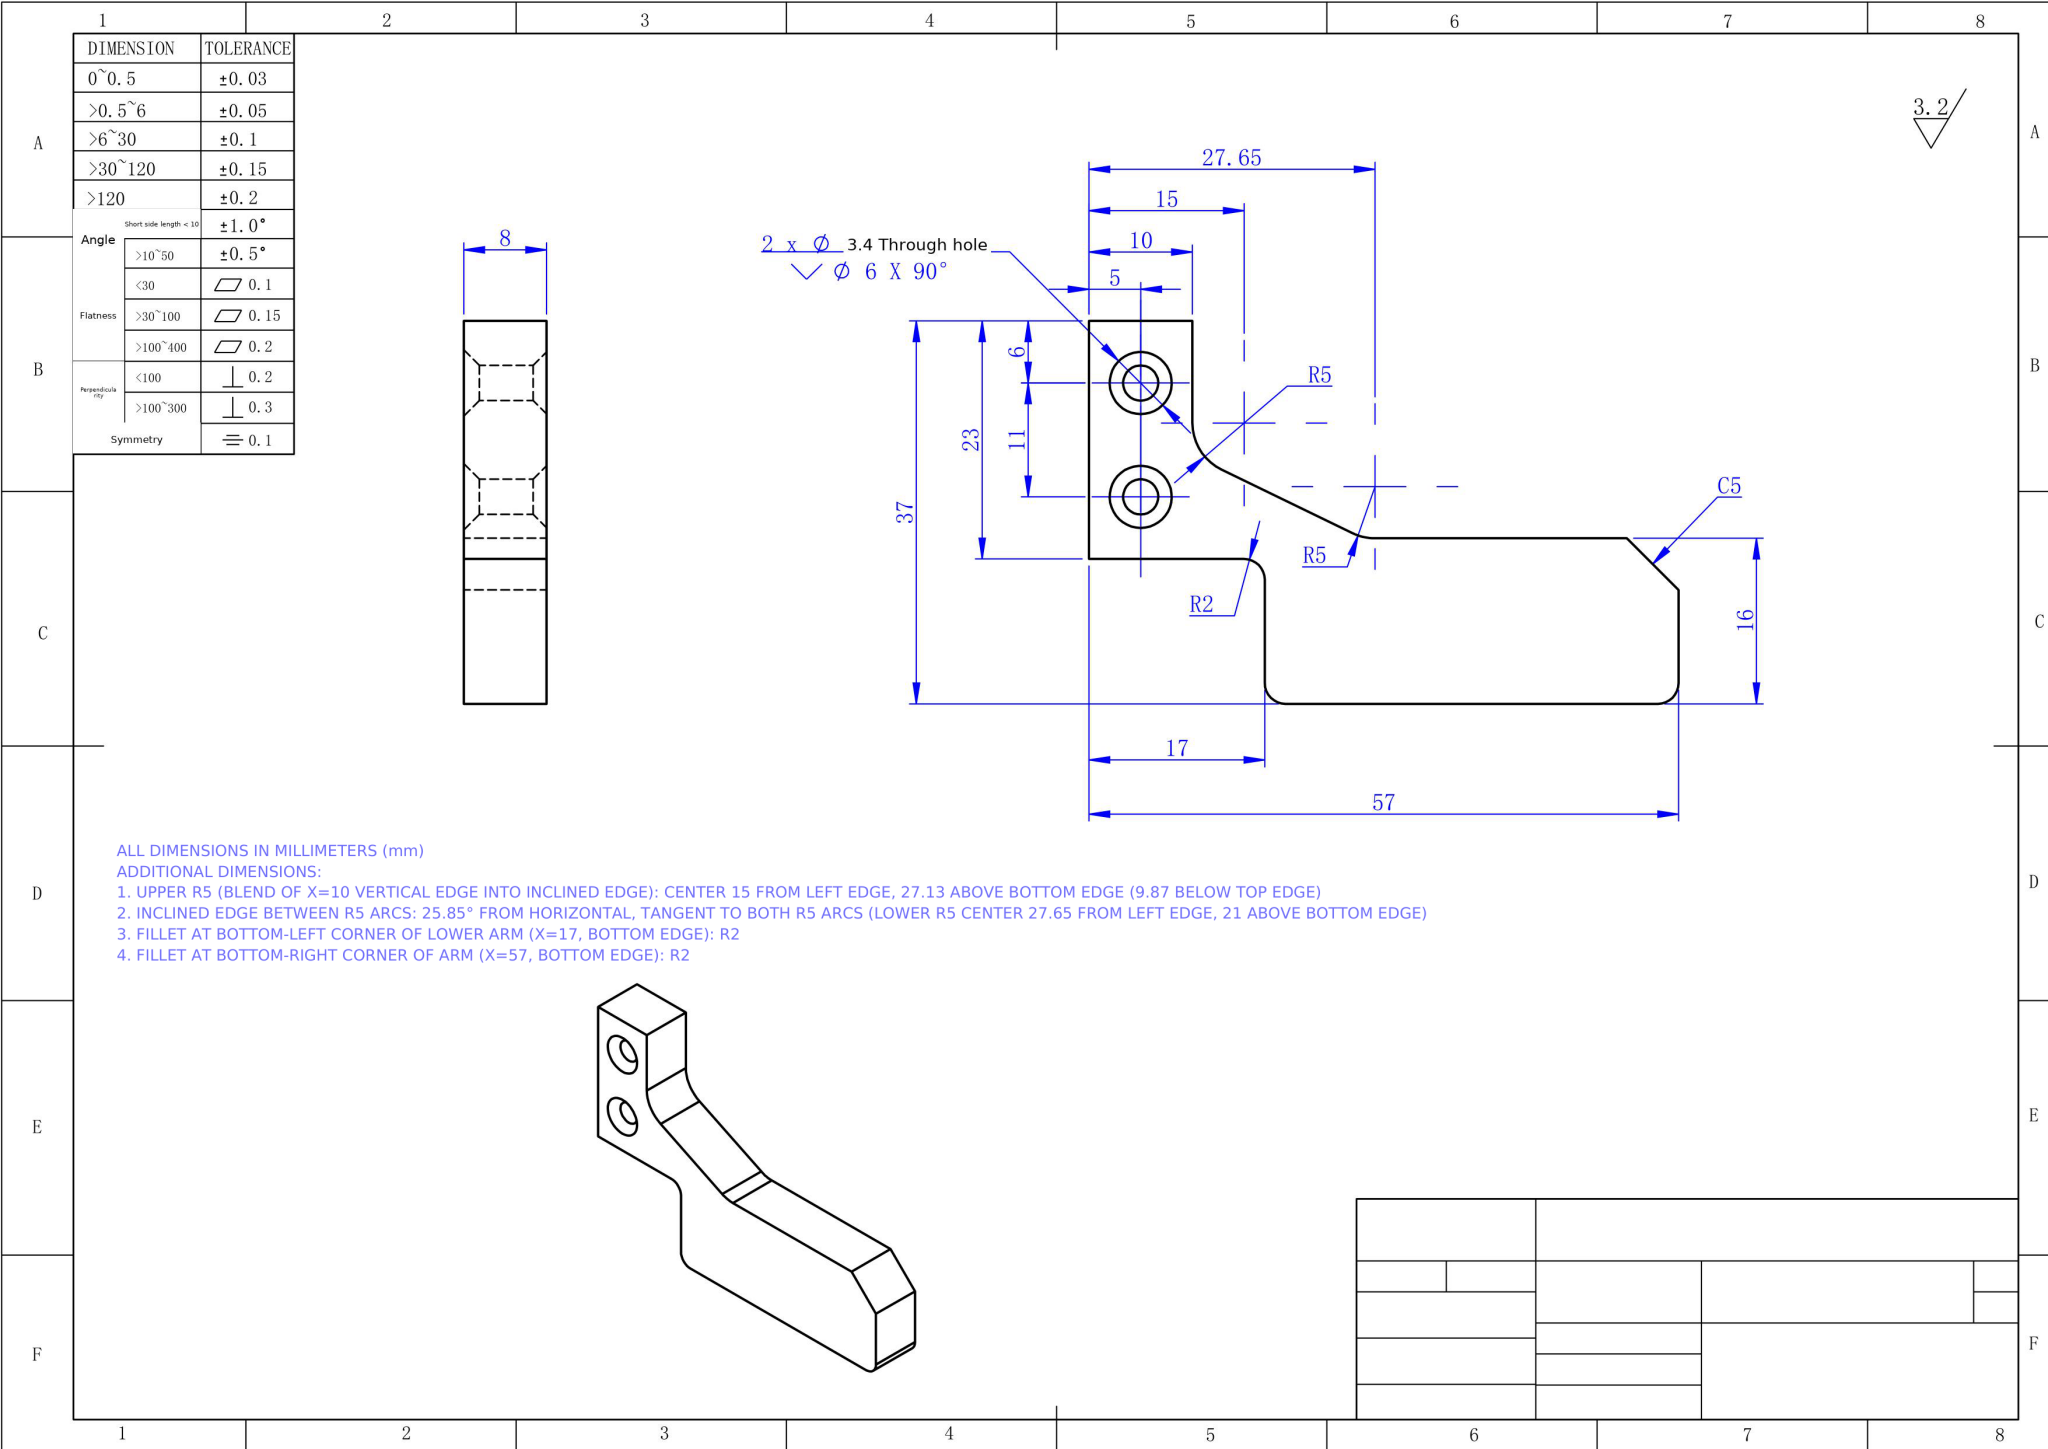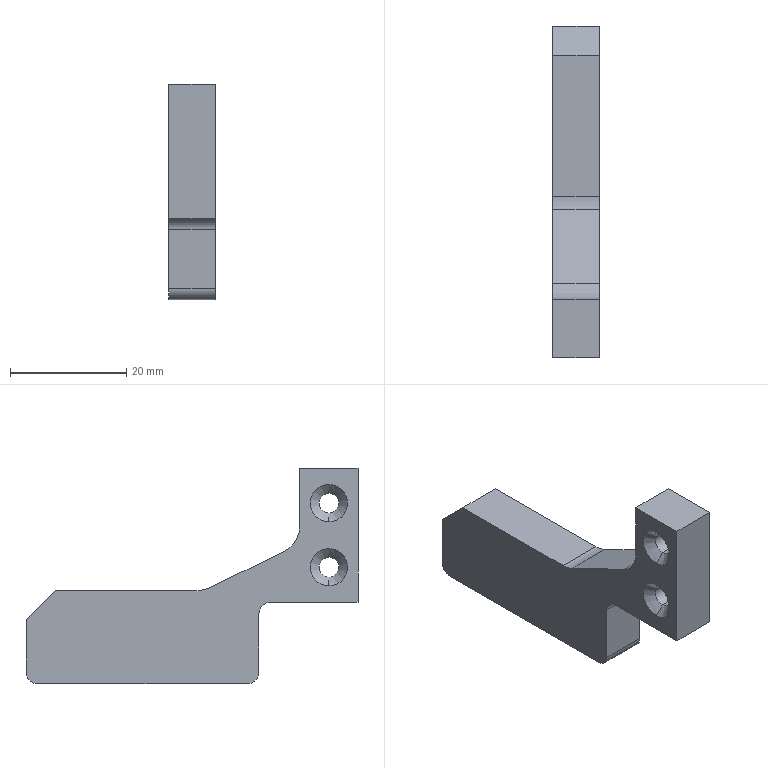Part | NX | mm | 1 solid | 29 faces | box 8 x 57 x 37 mm | volume 7308 mm3 | plane 12 | cylinder 9 | cone 8 | commonest cylinder face diameters 3.4 x4 4 x3 10 x2
STEP:
#1=COLOUR_RGB('',0.7529,0.7529,0.7529);
#2=FILL_AREA_STYLE_COLOUR('',#1);
#3=FILL_AREA_STYLE('',(#2));
#4=SURFACE_STYLE_FILL_AREA(#3);
#5=SURFACE_SIDE_STYLE('',(#4));
#6=SURFACE_STYLE_USAGE(.BOTH.,#5);
#7=PRESENTATION_STYLE_ASSIGNMENT((#6));
#8=CARTESIAN_POINT('',(1.5,5.,18.3));
#9=VERTEX_POINT('',#8);
#10=CARTESIAN_POINT('',(1.5,5.,21.7));
#11=VERTEX_POINT('',#10);
#12=CARTESIAN_POINT('',(1.5,5.,20.));
#13=DIRECTION('',(-1.,0.,0.));
#14=DIRECTION('',(0.,0.,1.));
#15=AXIS2_PLACEMENT_3D('',#12,#13,#14);
#16=CIRCLE('',#15,1.7);
#17=EDGE_CURVE('',#9,#11,#16,.T.);
#18=ORIENTED_EDGE('',*,*,#17,.F.);
#19=CARTESIAN_POINT('',(-0.,5.,16.8));
#20=VERTEX_POINT('',#19);
#21=CARTESIAN_POINT('',(-0.,5.,16.8));
#22=DIRECTION('',(-0.7071,0.,-0.7071));
#23=VECTOR('',#22,1000.);
#24=LINE('',#21,#23);
#25=EDGE_CURVE('',#9,#20,#24,.T.);
#26=ORIENTED_EDGE('',*,*,#25,.T.);
#27=CARTESIAN_POINT('',(-0.,5.,23.2));
#28=VERTEX_POINT('',#27);
#29=CARTESIAN_POINT('',(-0.,5.,20.));
#30=DIRECTION('',(-1.,0.,0.));
#31=DIRECTION('',(0.,0.,1.));
#32=AXIS2_PLACEMENT_3D('',#29,#30,#31);
#33=CIRCLE('',#32,3.2);
#34=EDGE_CURVE('',#20,#28,#33,.T.);
#35=ORIENTED_EDGE('',*,*,#34,.T.);
#36=CARTESIAN_POINT('',(-0.,5.,23.2));
#37=DIRECTION('',(-0.7071,0.,0.7071));
#38=VECTOR('',#37,1000.);
#39=LINE('',#36,#38);
#40=EDGE_CURVE('',#11,#28,#39,.T.);
#41=ORIENTED_EDGE('',*,*,#40,.F.);
#42=EDGE_LOOP('',(#18,#26,#35,#41));
#43=FACE_OUTER_BOUND('',#42,.T.);
#44=CARTESIAN_POINT('',(-0.,5.,20.));
#45=DIRECTION('',(-1.,0.,0.));
#46=DIRECTION('',(0.,0.,1.));
#47=AXIS2_PLACEMENT_3D('',#44,#45,#46);
#48=CONICAL_SURFACE('',#47,3.2,0.7854);
#49=ADVANCED_FACE('',(#43),#48,.F.);
#50=CARTESIAN_POINT('',(1.5,5.,29.3));
#51=VERTEX_POINT('',#50);
#52=CARTESIAN_POINT('',(1.5,5.,32.7));
#53=VERTEX_POINT('',#52);
#54=CARTESIAN_POINT('',(1.5,5.,31.));
#55=DIRECTION('',(-1.,0.,0.));
#56=DIRECTION('',(0.,0.,1.));
#57=AXIS2_PLACEMENT_3D('',#54,#55,#56);
#58=CIRCLE('',#57,1.7);
#59=EDGE_CURVE('',#51,#53,#58,.T.);
#60=ORIENTED_EDGE('',*,*,#59,.F.);
#61=CARTESIAN_POINT('',(-0.,5.,27.8));
#62=VERTEX_POINT('',#61);
#63=CARTESIAN_POINT('',(-0.,5.,27.8));
#64=DIRECTION('',(-0.7071,0.,-0.7071));
#65=VECTOR('',#64,1000.);
#66=LINE('',#63,#65);
#67=EDGE_CURVE('',#51,#62,#66,.T.);
#68=ORIENTED_EDGE('',*,*,#67,.T.);
#69=CARTESIAN_POINT('',(-0.,5.,34.2));
#70=VERTEX_POINT('',#69);
#71=CARTESIAN_POINT('',(-0.,5.,31.));
#72=DIRECTION('',(-1.,0.,0.));
#73=DIRECTION('',(0.,0.,1.));
#74=AXIS2_PLACEMENT_3D('',#71,#72,#73);
#75=CIRCLE('',#74,3.2);
#76=EDGE_CURVE('',#62,#70,#75,.T.);
#77=ORIENTED_EDGE('',*,*,#76,.T.);
#78=CARTESIAN_POINT('',(-0.,5.,34.2));
#79=DIRECTION('',(-0.7071,0.,0.7071));
#80=VECTOR('',#79,1000.);
#81=LINE('',#78,#80);
#82=EDGE_CURVE('',#53,#70,#81,.T.);
#83=ORIENTED_EDGE('',*,*,#82,.F.);
#84=EDGE_LOOP('',(#60,#68,#77,#83));
#85=FACE_OUTER_BOUND('',#84,.T.);
#86=CARTESIAN_POINT('',(-0.,5.,31.));
#87=DIRECTION('',(-1.,0.,0.));
#88=DIRECTION('',(0.,0.,1.));
#89=AXIS2_PLACEMENT_3D('',#86,#87,#88);
#90=CONICAL_SURFACE('',#89,3.2,0.7854);
#91=ADVANCED_FACE('',(#85),#90,.F.);
#92=CARTESIAN_POINT('',(6.7,5.,32.7));
#93=VERTEX_POINT('',#92);
#94=CARTESIAN_POINT('',(6.7,5.,29.3));
#95=VERTEX_POINT('',#94);
#96=CARTESIAN_POINT('',(6.7,5.,31.));
#97=DIRECTION('',(1.,0.,0.));
#98=DIRECTION('',(0.,0.,-1.));
#99=AXIS2_PLACEMENT_3D('',#96,#97,#98);
#100=CIRCLE('',#99,1.7);
#101=EDGE_CURVE('',#93,#95,#100,.T.);
#102=ORIENTED_EDGE('',*,*,#101,.F.);
#103=CARTESIAN_POINT('',(8.,5.,34.));
#104=VERTEX_POINT('',#103);
#105=CARTESIAN_POINT('',(8.,5.,34.));
#106=DIRECTION('',(0.7071,0.,0.7071));
#107=VECTOR('',#106,1000.);
#108=LINE('',#105,#107);
#109=EDGE_CURVE('',#93,#104,#108,.T.);
#110=ORIENTED_EDGE('',*,*,#109,.T.);
#111=CARTESIAN_POINT('',(8.,5.,28.));
#112=VERTEX_POINT('',#111);
#113=CARTESIAN_POINT('',(8.,5.,31.));
#114=DIRECTION('',(1.,0.,0.));
#115=DIRECTION('',(0.,0.,-1.));
#116=AXIS2_PLACEMENT_3D('',#113,#114,#115);
#117=CIRCLE('',#116,3.);
#118=EDGE_CURVE('',#104,#112,#117,.T.);
#119=ORIENTED_EDGE('',*,*,#118,.T.);
#120=CARTESIAN_POINT('',(8.,5.,28.));
#121=DIRECTION('',(0.7071,0.,-0.7071));
#122=VECTOR('',#121,1000.);
#123=LINE('',#120,#122);
#124=EDGE_CURVE('',#95,#112,#123,.T.);
#125=ORIENTED_EDGE('',*,*,#124,.F.);
#126=EDGE_LOOP('',(#102,#110,#119,#125));
#127=FACE_OUTER_BOUND('',#126,.T.);
#128=CARTESIAN_POINT('',(8.,5.,31.));
#129=DIRECTION('',(1.,0.,0.));
#130=DIRECTION('',(0.,0.,-1.));
#131=AXIS2_PLACEMENT_3D('',#128,#129,#130);
#132=CONICAL_SURFACE('',#131,3.,0.7854);
#133=ADVANCED_FACE('',(#127),#132,.F.);
#134=ORIENTED_EDGE('',*,*,#59,.T.);
#135=CARTESIAN_POINT('',(8.,5.,32.7));
#136=DIRECTION('',(1.,0.,0.));
#137=VECTOR('',#136,1000.);
#138=LINE('',#135,#137);
#139=EDGE_CURVE('',#53,#93,#138,.T.);
#140=ORIENTED_EDGE('',*,*,#139,.T.);
#141=ORIENTED_EDGE('',*,*,#101,.T.);
#142=CARTESIAN_POINT('',(8.,5.,29.3));
#143=DIRECTION('',(1.,0.,0.));
#144=VECTOR('',#143,1000.);
#145=LINE('',#142,#144);
#146=EDGE_CURVE('',#51,#95,#145,.T.);
#147=ORIENTED_EDGE('',*,*,#146,.F.);
#148=EDGE_LOOP('',(#134,#140,#141,#147));
#149=FACE_OUTER_BOUND('',#148,.T.);
#150=CARTESIAN_POINT('',(8.,5.,31.));
#151=DIRECTION('',(1.,0.,0.));
#152=DIRECTION('',(0.,0.,-1.));
#153=AXIS2_PLACEMENT_3D('',#150,#151,#152);
#154=CYLINDRICAL_SURFACE('',#153,1.7);
#155=ADVANCED_FACE('',(#149),#154,.F.);
#156=CARTESIAN_POINT('',(6.7,5.,21.7));
#157=VERTEX_POINT('',#156);
#158=CARTESIAN_POINT('',(6.7,5.,18.3));
#159=VERTEX_POINT('',#158);
#160=CARTESIAN_POINT('',(6.7,5.,20.));
#161=DIRECTION('',(1.,0.,0.));
#162=DIRECTION('',(0.,0.,-1.));
#163=AXIS2_PLACEMENT_3D('',#160,#161,#162);
#164=CIRCLE('',#163,1.7);
#165=EDGE_CURVE('',#157,#159,#164,.T.);
#166=ORIENTED_EDGE('',*,*,#165,.F.);
#167=CARTESIAN_POINT('',(8.,5.,23.));
#168=VERTEX_POINT('',#167);
#169=CARTESIAN_POINT('',(8.,5.,23.));
#170=DIRECTION('',(0.7071,0.,0.7071));
#171=VECTOR('',#170,1000.);
#172=LINE('',#169,#171);
#173=EDGE_CURVE('',#157,#168,#172,.T.);
#174=ORIENTED_EDGE('',*,*,#173,.T.);
#175=CARTESIAN_POINT('',(8.,5.,17.));
#176=VERTEX_POINT('',#175);
#177=CARTESIAN_POINT('',(8.,5.,20.));
#178=DIRECTION('',(1.,0.,0.));
#179=DIRECTION('',(0.,0.,-1.));
#180=AXIS2_PLACEMENT_3D('',#177,#178,#179);
#181=CIRCLE('',#180,3.);
#182=EDGE_CURVE('',#168,#176,#181,.T.);
#183=ORIENTED_EDGE('',*,*,#182,.T.);
#184=CARTESIAN_POINT('',(8.,5.,17.));
#185=DIRECTION('',(0.7071,0.,-0.7071));
#186=VECTOR('',#185,1000.);
#187=LINE('',#184,#186);
#188=EDGE_CURVE('',#159,#176,#187,.T.);
#189=ORIENTED_EDGE('',*,*,#188,.F.);
#190=EDGE_LOOP('',(#166,#174,#183,#189));
#191=FACE_OUTER_BOUND('',#190,.T.);
#192=CARTESIAN_POINT('',(8.,5.,20.));
#193=DIRECTION('',(1.,0.,0.));
#194=DIRECTION('',(0.,0.,-1.));
#195=AXIS2_PLACEMENT_3D('',#192,#193,#194);
#196=CONICAL_SURFACE('',#195,3.,0.7854);
#197=ADVANCED_FACE('',(#191),#196,.F.);
#198=ORIENTED_EDGE('',*,*,#17,.T.);
#199=CARTESIAN_POINT('',(8.,5.,21.7));
#200=DIRECTION('',(1.,0.,0.));
#201=VECTOR('',#200,1000.);
#202=LINE('',#199,#201);
#203=EDGE_CURVE('',#11,#157,#202,.T.);
#204=ORIENTED_EDGE('',*,*,#203,.T.);
#205=ORIENTED_EDGE('',*,*,#165,.T.);
#206=CARTESIAN_POINT('',(8.,5.,18.3));
#207=DIRECTION('',(1.,0.,0.));
#208=VECTOR('',#207,1000.);
#209=LINE('',#206,#208);
#210=EDGE_CURVE('',#9,#159,#209,.T.);
#211=ORIENTED_EDGE('',*,*,#210,.F.);
#212=EDGE_LOOP('',(#198,#204,#205,#211));
#213=FACE_OUTER_BOUND('',#212,.T.);
#214=CARTESIAN_POINT('',(8.,5.,20.));
#215=DIRECTION('',(1.,0.,0.));
#216=DIRECTION('',(0.,0.,-1.));
#217=AXIS2_PLACEMENT_3D('',#214,#215,#216);
#218=CYLINDRICAL_SURFACE('',#217,1.7);
#219=ADVANCED_FACE('',(#213),#218,.F.);
#220=CARTESIAN_POINT('',(-0.,5.,20.));
#221=DIRECTION('',(-1.,0.,0.));
#222=DIRECTION('',(0.,0.,1.));
#223=AXIS2_PLACEMENT_3D('',#220,#221,#222);
#224=CIRCLE('',#223,3.2);
#225=EDGE_CURVE('',#28,#20,#224,.T.);
#226=ORIENTED_EDGE('',*,*,#225,.F.);
#227=ORIENTED_EDGE('',*,*,#34,.F.);
#228=EDGE_LOOP('',(#226,#227));
#229=FACE_BOUND('',#228,.T.);
#230=CARTESIAN_POINT('',(-0.,5.,31.));
#231=DIRECTION('',(-1.,0.,0.));
#232=DIRECTION('',(0.,0.,1.));
#233=AXIS2_PLACEMENT_3D('',#230,#231,#232);
#234=CIRCLE('',#233,3.2);
#235=EDGE_CURVE('',#70,#62,#234,.T.);
#236=ORIENTED_EDGE('',*,*,#235,.F.);
#237=ORIENTED_EDGE('',*,*,#76,.F.);
#238=EDGE_LOOP('',(#236,#237));
#239=FACE_BOUND('',#238,.T.);
#240=CARTESIAN_POINT('',(-0.,10.,27.132));
#241=VERTEX_POINT('',#240);
#242=CARTESIAN_POINT('',(-0.,10.,37.));
#243=VERTEX_POINT('',#242);
#244=CARTESIAN_POINT('',(-0.,10.,42.));
#245=DIRECTION('',(-0.,0.,1.));
#246=VECTOR('',#245,1000.);
#247=LINE('',#244,#246);
#248=EDGE_CURVE('',#241,#243,#247,.T.);
#249=ORIENTED_EDGE('',*,*,#248,.F.);
#250=CARTESIAN_POINT('',(-0.,12.819,22.633));
#251=VERTEX_POINT('',#250);
#252=CARTESIAN_POINT('',(-0.,15.,27.132));
#253=DIRECTION('',(1.,0.,0.));
#254=DIRECTION('',(-0.,1.,0.));
#255=AXIS2_PLACEMENT_3D('',#252,#253,#254);
#256=CIRCLE('',#255,5.);
#257=EDGE_CURVE('',#241,#251,#256,.T.);
#258=ORIENTED_EDGE('',*,*,#257,.T.);
#259=CARTESIAN_POINT('',(-0.,25.467,16.501));
#260=VERTEX_POINT('',#259);
#261=CARTESIAN_POINT('',(-0.,26.5,16.));
#262=DIRECTION('',(0.,-0.8998,0.4363));
#263=VECTOR('',#262,1000.);
#264=LINE('',#261,#263);
#265=EDGE_CURVE('',#260,#251,#264,.T.);
#266=ORIENTED_EDGE('',*,*,#265,.F.);
#267=CARTESIAN_POINT('',(-0.,27.648,16.));
#268=VERTEX_POINT('',#267);
#269=CARTESIAN_POINT('',(-0.,27.648,21.));
#270=DIRECTION('',(1.,0.,0.));
#271=DIRECTION('',(-0.,1.,0.));
#272=AXIS2_PLACEMENT_3D('',#269,#270,#271);
#273=CIRCLE('',#272,5.);
#274=EDGE_CURVE('',#260,#268,#273,.T.);
#275=ORIENTED_EDGE('',*,*,#274,.T.);
#276=CARTESIAN_POINT('',(-0.,52.,16.));
#277=VERTEX_POINT('',#276);
#278=CARTESIAN_POINT('',(-0.,0.,16.));
#279=DIRECTION('',(-0.,1.,0.));
#280=VECTOR('',#279,1000.);
#281=LINE('',#278,#280);
#282=EDGE_CURVE('',#268,#277,#281,.T.);
#283=ORIENTED_EDGE('',*,*,#282,.T.);
#284=CARTESIAN_POINT('',(-0.,57.,11.));
#285=VERTEX_POINT('',#284);
#286=CARTESIAN_POINT('',(-0.,57.,11.));
#287=DIRECTION('',(-0.,0.7071,-0.7071));
#288=VECTOR('',#287,1000.);
#289=LINE('',#286,#288);
#290=EDGE_CURVE('',#277,#285,#289,.T.);
#291=ORIENTED_EDGE('',*,*,#290,.T.);
#292=CARTESIAN_POINT('',(-0.,57.,2.));
#293=VERTEX_POINT('',#292);
#294=CARTESIAN_POINT('',(-0.,57.,42.));
#295=DIRECTION('',(0.,0.,-1.));
#296=VECTOR('',#295,1000.);
#297=LINE('',#294,#296);
#298=EDGE_CURVE('',#285,#293,#297,.T.);
#299=ORIENTED_EDGE('',*,*,#298,.T.);
#300=CARTESIAN_POINT('',(-0.,55.,0.));
#301=VERTEX_POINT('',#300);
#302=CARTESIAN_POINT('',(-0.,55.,2.));
#303=DIRECTION('',(-1.,-0.,0.));
#304=DIRECTION('',(-0.,1.,0.));
#305=AXIS2_PLACEMENT_3D('',#302,#303,#304);
#306=CIRCLE('',#305,2.);
#307=EDGE_CURVE('',#293,#301,#306,.T.);
#308=ORIENTED_EDGE('',*,*,#307,.T.);
#309=CARTESIAN_POINT('',(-0.,19.,0.));
#310=VERTEX_POINT('',#309);
#311=CARTESIAN_POINT('',(0.,0.,0.));
#312=DIRECTION('',(0.,-1.,0.));
#313=VECTOR('',#312,1000.);
#314=LINE('',#311,#313);
#315=EDGE_CURVE('',#301,#310,#314,.T.);
#316=ORIENTED_EDGE('',*,*,#315,.T.);
#317=CARTESIAN_POINT('',(-0.,17.,2.));
#318=VERTEX_POINT('',#317);
#319=CARTESIAN_POINT('',(-0.,19.,2.));
#320=DIRECTION('',(-1.,-0.,0.));
#321=DIRECTION('',(-0.,1.,0.));
#322=AXIS2_PLACEMENT_3D('',#319,#320,#321);
#323=CIRCLE('',#322,2.);
#324=EDGE_CURVE('',#310,#318,#323,.T.);
#325=ORIENTED_EDGE('',*,*,#324,.T.);
#326=CARTESIAN_POINT('',(-0.,17.,12.));
#327=VERTEX_POINT('',#326);
#328=CARTESIAN_POINT('',(-0.,17.,14.));
#329=DIRECTION('',(0.,-0.,-1.));
#330=VECTOR('',#329,1000.);
#331=LINE('',#328,#330);
#332=EDGE_CURVE('',#327,#318,#331,.T.);
#333=ORIENTED_EDGE('',*,*,#332,.F.);
#334=CARTESIAN_POINT('',(-0.,15.,14.));
#335=VERTEX_POINT('',#334);
#336=CARTESIAN_POINT('',(-0.,15.,12.));
#337=DIRECTION('',(1.,0.,0.));
#338=DIRECTION('',(-0.,1.,0.));
#339=AXIS2_PLACEMENT_3D('',#336,#337,#338);
#340=CIRCLE('',#339,2.);
#341=EDGE_CURVE('',#327,#335,#340,.T.);
#342=ORIENTED_EDGE('',*,*,#341,.T.);
#343=CARTESIAN_POINT('',(-0.,-0.,14.));
#344=VERTEX_POINT('',#343);
#345=CARTESIAN_POINT('',(-0.,7.,14.));
#346=DIRECTION('',(-0.,1.,0.));
#347=VECTOR('',#346,1000.);
#348=LINE('',#345,#347);
#349=EDGE_CURVE('',#344,#335,#348,.T.);
#350=ORIENTED_EDGE('',*,*,#349,.F.);
#351=CARTESIAN_POINT('',(0.,-0.,37.));
#352=VERTEX_POINT('',#351);
#353=CARTESIAN_POINT('',(0.,-0.,14.));
#354=DIRECTION('',(-0.,0.,1.));
#355=VECTOR('',#354,1000.);
#356=LINE('',#353,#355);
#357=EDGE_CURVE('',#344,#352,#356,.T.);
#358=ORIENTED_EDGE('',*,*,#357,.T.);
#359=CARTESIAN_POINT('',(-0.,8.5,37.));
#360=DIRECTION('',(-0.,1.,0.));
#361=VECTOR('',#360,1000.);
#362=LINE('',#359,#361);
#363=EDGE_CURVE('',#352,#243,#362,.T.);
#364=ORIENTED_EDGE('',*,*,#363,.T.);
#365=EDGE_LOOP('',(#249,#258,#266,#275,#283,#291,#299,#308,#316,#325,#333,#342,#350,#358,#364));
#366=FACE_OUTER_BOUND('',#365,.T.);
#367=CARTESIAN_POINT('',(0.,0.,42.));
#368=DIRECTION('',(1.,0.,0.));
#369=DIRECTION('',(-0.,1.,0.));
#370=AXIS2_PLACEMENT_3D('',#367,#368,#369);
#371=PLANE('',#370);
#372=ADVANCED_FACE('',(#229,#239,#366),#371,.F.);
#373=CARTESIAN_POINT('',(8.,5.,31.));
#374=DIRECTION('',(1.,0.,0.));
#375=DIRECTION('',(0.,0.,-1.));
#376=AXIS2_PLACEMENT_3D('',#373,#374,#375);
#377=CIRCLE('',#376,3.);
#378=EDGE_CURVE('',#112,#104,#377,.T.);
#379=ORIENTED_EDGE('',*,*,#378,.F.);
#380=ORIENTED_EDGE('',*,*,#118,.F.);
#381=EDGE_LOOP('',(#379,#380));
#382=FACE_BOUND('',#381,.T.);
#383=CARTESIAN_POINT('',(8.,5.,20.));
#384=DIRECTION('',(1.,0.,0.));
#385=DIRECTION('',(0.,0.,-1.));
#386=AXIS2_PLACEMENT_3D('',#383,#384,#385);
#387=CIRCLE('',#386,3.);
#388=EDGE_CURVE('',#176,#168,#387,.T.);
#389=ORIENTED_EDGE('',*,*,#388,.F.);
#390=ORIENTED_EDGE('',*,*,#182,.F.);
#391=EDGE_LOOP('',(#389,#390));
#392=FACE_BOUND('',#391,.T.);
#393=CARTESIAN_POINT('',(8.,27.648,16.));
#394=VERTEX_POINT('',#393);
#395=CARTESIAN_POINT('',(8.,52.,16.));
#396=VERTEX_POINT('',#395);
#397=CARTESIAN_POINT('',(8.,79.315,16.));
#398=DIRECTION('',(-0.,1.,0.));
#399=VECTOR('',#398,1000.);
#400=LINE('',#397,#399);
#401=EDGE_CURVE('',#394,#396,#400,.T.);
#402=ORIENTED_EDGE('',*,*,#401,.F.);
#403=CARTESIAN_POINT('',(8.,25.467,16.501));
#404=VERTEX_POINT('',#403);
#405=CARTESIAN_POINT('',(8.,27.648,21.));
#406=DIRECTION('',(-1.,-0.,0.));
#407=DIRECTION('',(0.,-1.,0.));
#408=AXIS2_PLACEMENT_3D('',#405,#406,#407);
#409=CIRCLE('',#408,5.);
#410=EDGE_CURVE('',#394,#404,#409,.T.);
#411=ORIENTED_EDGE('',*,*,#410,.T.);
#412=CARTESIAN_POINT('',(8.,12.819,22.633));
#413=VERTEX_POINT('',#412);
#414=CARTESIAN_POINT('',(8.,26.5,16.));
#415=DIRECTION('',(0.,-0.8998,0.4363));
#416=VECTOR('',#415,1000.);
#417=LINE('',#414,#416);
#418=EDGE_CURVE('',#404,#413,#417,.T.);
#419=ORIENTED_EDGE('',*,*,#418,.T.);
#420=CARTESIAN_POINT('',(8.,10.,27.132));
#421=VERTEX_POINT('',#420);
#422=CARTESIAN_POINT('',(8.,15.,27.132));
#423=DIRECTION('',(-1.,-0.,0.));
#424=DIRECTION('',(0.,-1.,0.));
#425=AXIS2_PLACEMENT_3D('',#422,#423,#424);
#426=CIRCLE('',#425,5.);
#427=EDGE_CURVE('',#413,#421,#426,.T.);
#428=ORIENTED_EDGE('',*,*,#427,.T.);
#429=CARTESIAN_POINT('',(8.,10.,37.));
#430=VERTEX_POINT('',#429);
#431=CARTESIAN_POINT('',(8.,10.,42.));
#432=DIRECTION('',(-0.,0.,1.));
#433=VECTOR('',#432,1000.);
#434=LINE('',#431,#433);
#435=EDGE_CURVE('',#421,#430,#434,.T.);
#436=ORIENTED_EDGE('',*,*,#435,.T.);
#437=CARTESIAN_POINT('',(8.,-0.,37.));
#438=VERTEX_POINT('',#437);
#439=CARTESIAN_POINT('',(8.,8.5,37.));
#440=DIRECTION('',(0.,-1.,0.));
#441=VECTOR('',#440,1000.);
#442=LINE('',#439,#441);
#443=EDGE_CURVE('',#430,#438,#442,.T.);
#444=ORIENTED_EDGE('',*,*,#443,.T.);
#445=CARTESIAN_POINT('',(8.,-0.,14.));
#446=VERTEX_POINT('',#445);
#447=CARTESIAN_POINT('',(8.,-0.,14.));
#448=DIRECTION('',(0.,-0.,-1.));
#449=VECTOR('',#448,1000.);
#450=LINE('',#447,#449);
#451=EDGE_CURVE('',#438,#446,#450,.T.);
#452=ORIENTED_EDGE('',*,*,#451,.T.);
#453=CARTESIAN_POINT('',(8.,15.,14.));
#454=VERTEX_POINT('',#453);
#455=CARTESIAN_POINT('',(8.,0.,14.));
#456=DIRECTION('',(-0.,1.,0.));
#457=VECTOR('',#456,1000.);
#458=LINE('',#455,#457);
#459=EDGE_CURVE('',#446,#454,#458,.T.);
#460=ORIENTED_EDGE('',*,*,#459,.T.);
#461=CARTESIAN_POINT('',(8.,17.,12.));
#462=VERTEX_POINT('',#461);
#463=CARTESIAN_POINT('',(8.,15.,12.));
#464=DIRECTION('',(-1.,-0.,0.));
#465=DIRECTION('',(0.,-1.,0.));
#466=AXIS2_PLACEMENT_3D('',#463,#464,#465);
#467=CIRCLE('',#466,2.);
#468=EDGE_CURVE('',#454,#462,#467,.T.);
#469=ORIENTED_EDGE('',*,*,#468,.T.);
#470=CARTESIAN_POINT('',(8.,17.,2.));
#471=VERTEX_POINT('',#470);
#472=CARTESIAN_POINT('',(8.,17.,42.));
#473=DIRECTION('',(0.,-0.,-1.));
#474=VECTOR('',#473,1000.);
#475=LINE('',#472,#474);
#476=EDGE_CURVE('',#462,#471,#475,.T.);
#477=ORIENTED_EDGE('',*,*,#476,.T.);
#478=CARTESIAN_POINT('',(8.,19.,0.));
#479=VERTEX_POINT('',#478);
#480=CARTESIAN_POINT('',(8.,19.,2.));
#481=DIRECTION('',(1.,0.,0.));
#482=DIRECTION('',(0.,-1.,0.));
#483=AXIS2_PLACEMENT_3D('',#480,#481,#482);
#484=CIRCLE('',#483,2.);
#485=EDGE_CURVE('',#471,#479,#484,.T.);
#486=ORIENTED_EDGE('',*,*,#485,.T.);
#487=CARTESIAN_POINT('',(8.,55.,0.));
#488=VERTEX_POINT('',#487);
#489=CARTESIAN_POINT('',(8.,0.,0.));
#490=DIRECTION('',(-0.,1.,0.));
#491=VECTOR('',#490,1000.);
#492=LINE('',#489,#491);
#493=EDGE_CURVE('',#479,#488,#492,.T.);
#494=ORIENTED_EDGE('',*,*,#493,.T.);
#495=CARTESIAN_POINT('',(8.,57.,2.));
#496=VERTEX_POINT('',#495);
#497=CARTESIAN_POINT('',(8.,55.,2.));
#498=DIRECTION('',(1.,0.,0.));
#499=DIRECTION('',(0.,-1.,0.));
#500=AXIS2_PLACEMENT_3D('',#497,#498,#499);
#501=CIRCLE('',#500,2.);
#502=EDGE_CURVE('',#488,#496,#501,.T.);
#503=ORIENTED_EDGE('',*,*,#502,.T.);
#504=CARTESIAN_POINT('',(8.,57.,11.));
#505=VERTEX_POINT('',#504);
#506=CARTESIAN_POINT('',(8.,57.,42.));
#507=DIRECTION('',(0.,0.,-1.));
#508=VECTOR('',#507,1000.);
#509=LINE('',#506,#508);
#510=EDGE_CURVE('',#505,#496,#509,.T.);
#511=ORIENTED_EDGE('',*,*,#510,.F.);
#512=CARTESIAN_POINT('',(8.,57.,11.));
#513=DIRECTION('',(0.,-0.7071,0.7071));
#514=VECTOR('',#513,1000.);
#515=LINE('',#512,#514);
#516=EDGE_CURVE('',#505,#396,#515,.T.);
#517=ORIENTED_EDGE('',*,*,#516,.T.);
#518=EDGE_LOOP('',(#402,#411,#419,#428,#436,#444,#452,#460,#469,#477,#486,#494,#503,#511,#517));
#519=FACE_OUTER_BOUND('',#518,.T.);
#520=CARTESIAN_POINT('',(8.,0.,42.));
#521=DIRECTION('',(-1.,-0.,0.));
#522=DIRECTION('',(0.,-1.,0.));
#523=AXIS2_PLACEMENT_3D('',#520,#521,#522);
#524=PLANE('',#523);
#525=ADVANCED_FACE('',(#382,#392,#519),#524,.F.);
#526=ORIENTED_EDGE('',*,*,#510,.T.);
#527=CARTESIAN_POINT('',(-0.,57.,2.));
#528=DIRECTION('',(-1.,0.,0.));
#529=VECTOR('',#528,1000.);
#530=LINE('',#527,#529);
#531=EDGE_CURVE('',#496,#293,#530,.T.);
#532=ORIENTED_EDGE('',*,*,#531,.T.);
#533=ORIENTED_EDGE('',*,*,#298,.F.);
#534=CARTESIAN_POINT('',(-0.,57.,11.));
#535=DIRECTION('',(1.,0.,-0.));
#536=VECTOR('',#535,1000.);
#537=LINE('',#534,#536);
#538=EDGE_CURVE('',#285,#505,#537,.T.);
#539=ORIENTED_EDGE('',*,*,#538,.T.);
#540=EDGE_LOOP('',(#526,#532,#533,#539));
#541=FACE_OUTER_BOUND('',#540,.T.);
#542=CARTESIAN_POINT('',(-0.,57.,42.));
#543=DIRECTION('',(0.,-1.,0.));
#544=DIRECTION('',(0.,0.,-1.));
#545=AXIS2_PLACEMENT_3D('',#542,#543,#544);
#546=PLANE('',#545);
#547=ADVANCED_FACE('',(#541),#546,.F.);
#548=ORIENTED_EDGE('',*,*,#493,.F.);
#549=CARTESIAN_POINT('',(-0.,19.,0.));
#550=DIRECTION('',(-1.,-0.,0.));
#551=VECTOR('',#550,1000.);
#552=LINE('',#549,#551);
#553=EDGE_CURVE('',#479,#310,#552,.T.);
#554=ORIENTED_EDGE('',*,*,#553,.T.);
#555=ORIENTED_EDGE('',*,*,#315,.F.);
#556=CARTESIAN_POINT('',(8.,55.,0.));
#557=DIRECTION('',(1.,0.,0.));
#558=VECTOR('',#557,1000.);
#559=LINE('',#556,#558);
#560=EDGE_CURVE('',#301,#488,#559,.T.);
#561=ORIENTED_EDGE('',*,*,#560,.T.);
#562=EDGE_LOOP('',(#548,#554,#555,#561));
#563=FACE_OUTER_BOUND('',#562,.T.);
#564=CARTESIAN_POINT('',(0.,0.,0.));
#565=DIRECTION('',(0.,0.,-1.));
#566=DIRECTION('',(-1.,0.,0.));
#567=AXIS2_PLACEMENT_3D('',#564,#565,#566);
#568=PLANE('',#567);
#569=ADVANCED_FACE('',(#563),#568,.T.);
#570=ORIENTED_EDGE('',*,*,#282,.F.);
#571=CARTESIAN_POINT('',(8.,27.648,16.));
#572=DIRECTION('',(1.,0.,-0.));
#573=VECTOR('',#572,1000.);
#574=LINE('',#571,#573);
#575=EDGE_CURVE('',#268,#394,#574,.T.);
#576=ORIENTED_EDGE('',*,*,#575,.T.);
#577=ORIENTED_EDGE('',*,*,#401,.T.);
#578=CARTESIAN_POINT('',(-2.,52.,16.));
#579=DIRECTION('',(-1.,0.,0.));
#580=VECTOR('',#579,1000.);
#581=LINE('',#578,#580);
#582=EDGE_CURVE('',#396,#277,#581,.T.);
#583=ORIENTED_EDGE('',*,*,#582,.T.);
#584=EDGE_LOOP('',(#570,#576,#577,#583));
#585=FACE_OUTER_BOUND('',#584,.T.);
#586=CARTESIAN_POINT('',(-2.,79.315,16.));
#587=DIRECTION('',(-0.,0.,-1.));
#588=DIRECTION('',(0.,1.,0.));
#589=AXIS2_PLACEMENT_3D('',#586,#587,#588);
#590=PLANE('',#589);
#591=ADVANCED_FACE('',(#585),#590,.F.);
#592=ORIENTED_EDGE('',*,*,#290,.F.);
#593=ORIENTED_EDGE('',*,*,#582,.F.);
#594=ORIENTED_EDGE('',*,*,#516,.F.);
#595=ORIENTED_EDGE('',*,*,#538,.F.);
#596=EDGE_LOOP('',(#592,#593,#594,#595));
#597=FACE_OUTER_BOUND('',#596,.T.);
#598=CARTESIAN_POINT('',(-0.,57.,11.));
#599=DIRECTION('',(-0.,-0.7071,-0.7071));
#600=DIRECTION('',(1.,0.,-0.));
#601=AXIS2_PLACEMENT_3D('',#598,#599,#600);
#602=PLANE('',#601);
#603=ADVANCED_FACE('',(#597),#602,.F.);
#604=ORIENTED_EDGE('',*,*,#476,.F.);
#605=CARTESIAN_POINT('',(-0.,17.,12.));
#606=DIRECTION('',(-1.,-0.,0.));
#607=VECTOR('',#606,1000.);
#608=LINE('',#605,#607);
#609=EDGE_CURVE('',#462,#327,#608,.T.);
#610=ORIENTED_EDGE('',*,*,#609,.T.);
#611=ORIENTED_EDGE('',*,*,#332,.T.);
#612=CARTESIAN_POINT('',(8.,17.,2.));
#613=DIRECTION('',(1.,0.,0.));
#614=VECTOR('',#613,1000.);
#615=LINE('',#612,#614);
#616=EDGE_CURVE('',#318,#471,#615,.T.);
#617=ORIENTED_EDGE('',*,*,#616,.T.);
#618=EDGE_LOOP('',(#604,#610,#611,#617));
#619=FACE_OUTER_BOUND('',#618,.T.);
#620=CARTESIAN_POINT('',(10.,17.,14.));
#621=DIRECTION('',(-0.,1.,-0.));
#622=DIRECTION('',(0.,0.,1.));
#623=AXIS2_PLACEMENT_3D('',#620,#621,#622);
#624=PLANE('',#623);
#625=ADVANCED_FACE('',(#619),#624,.F.);
#626=ORIENTED_EDGE('',*,*,#459,.F.);
#627=CARTESIAN_POINT('',(32.52,-0.,14.));
#628=DIRECTION('',(-1.,-0.,0.));
#629=VECTOR('',#628,1000.);
#630=LINE('',#627,#629);
#631=EDGE_CURVE('',#446,#344,#630,.T.);
#632=ORIENTED_EDGE('',*,*,#631,.T.);
#633=ORIENTED_EDGE('',*,*,#349,.T.);
#634=CARTESIAN_POINT('',(8.,15.,14.));
#635=DIRECTION('',(1.,0.,0.));
#636=VECTOR('',#635,1000.);
#637=LINE('',#634,#636);
#638=EDGE_CURVE('',#335,#454,#637,.T.);
#639=ORIENTED_EDGE('',*,*,#638,.T.);
#640=EDGE_LOOP('',(#626,#632,#633,#639));
#641=FACE_OUTER_BOUND('',#640,.T.);
#642=CARTESIAN_POINT('',(10.,7.,14.));
#643=DIRECTION('',(0.,0.,1.));
#644=DIRECTION('',(1.,0.,0.));
#645=AXIS2_PLACEMENT_3D('',#642,#643,#644);
#646=PLANE('',#645);
#647=ADVANCED_FACE('',(#641),#646,.F.);
#648=ORIENTED_EDGE('',*,*,#443,.F.);
#649=CARTESIAN_POINT('',(10.,10.,37.));
#650=DIRECTION('',(1.,0.,0.));
#651=VECTOR('',#650,1000.);
#652=LINE('',#649,#651);
#653=EDGE_CURVE('',#243,#430,#652,.T.);
#654=ORIENTED_EDGE('',*,*,#653,.F.);
#655=ORIENTED_EDGE('',*,*,#363,.F.);
#656=CARTESIAN_POINT('',(32.52,-0.,37.));
#657=DIRECTION('',(-1.,-0.,0.));
#658=VECTOR('',#657,1000.);
#659=LINE('',#656,#658);
#660=EDGE_CURVE('',#438,#352,#659,.T.);
#661=ORIENTED_EDGE('',*,*,#660,.F.);
#662=EDGE_LOOP('',(#648,#654,#655,#661));
#663=FACE_OUTER_BOUND('',#662,.T.);
#664=CARTESIAN_POINT('',(32.52,8.5,37.));
#665=DIRECTION('',(0.,0.,1.));
#666=DIRECTION('',(1.,0.,0.));
#667=AXIS2_PLACEMENT_3D('',#664,#665,#666);
#668=PLANE('',#667);
#669=ADVANCED_FACE('',(#663),#668,.T.);
#670=ORIENTED_EDGE('',*,*,#631,.F.);
#671=ORIENTED_EDGE('',*,*,#451,.F.);
#672=ORIENTED_EDGE('',*,*,#660,.T.);
#673=ORIENTED_EDGE('',*,*,#357,.F.);
#674=EDGE_LOOP('',(#670,#671,#672,#673));
#675=FACE_OUTER_BOUND('',#674,.T.);
#676=CARTESIAN_POINT('',(32.52,-0.,14.));
#677=DIRECTION('',(0.,-1.,0.));
#678=DIRECTION('',(1.,0.,0.));
#679=AXIS2_PLACEMENT_3D('',#676,#677,#678);
#680=PLANE('',#679);
#681=ADVANCED_FACE('',(#675),#680,.T.);
#682=ORIENTED_EDGE('',*,*,#435,.F.);
#683=CARTESIAN_POINT('',(-0.,10.,27.132));
#684=DIRECTION('',(-1.,-0.,0.));
#685=VECTOR('',#684,1000.);
#686=LINE('',#683,#685);
#687=EDGE_CURVE('',#421,#241,#686,.T.);
#688=ORIENTED_EDGE('',*,*,#687,.T.);
#689=ORIENTED_EDGE('',*,*,#248,.T.);
#690=ORIENTED_EDGE('',*,*,#653,.T.);
#691=EDGE_LOOP('',(#682,#688,#689,#690));
#692=FACE_OUTER_BOUND('',#691,.T.);
#693=CARTESIAN_POINT('',(10.,10.,42.));
#694=DIRECTION('',(0.,-1.,0.));
#695=DIRECTION('',(1.,0.,0.));
#696=AXIS2_PLACEMENT_3D('',#693,#694,#695);
#697=PLANE('',#696);
#698=ADVANCED_FACE('',(#692),#697,.F.);
#699=ORIENTED_EDGE('',*,*,#203,.F.);
#700=CARTESIAN_POINT('',(1.5,5.,20.));
#701=DIRECTION('',(-1.,0.,0.));
#702=DIRECTION('',(0.,0.,1.));
#703=AXIS2_PLACEMENT_3D('',#700,#701,#702);
#704=CIRCLE('',#703,1.7);
#705=EDGE_CURVE('',#11,#9,#704,.T.);
#706=ORIENTED_EDGE('',*,*,#705,.T.);
#707=ORIENTED_EDGE('',*,*,#210,.T.);
#708=CARTESIAN_POINT('',(6.7,5.,20.));
#709=DIRECTION('',(1.,0.,0.));
#710=DIRECTION('',(0.,0.,-1.));
#711=AXIS2_PLACEMENT_3D('',#708,#709,#710);
#712=CIRCLE('',#711,1.7);
#713=EDGE_CURVE('',#159,#157,#712,.T.);
#714=ORIENTED_EDGE('',*,*,#713,.T.);
#715=EDGE_LOOP('',(#699,#706,#707,#714));
#716=FACE_OUTER_BOUND('',#715,.T.);
#717=CARTESIAN_POINT('',(8.,5.,20.));
#718=DIRECTION('',(1.,0.,0.));
#719=DIRECTION('',(0.,0.,-1.));
#720=AXIS2_PLACEMENT_3D('',#717,#718,#719);
#721=CYLINDRICAL_SURFACE('',#720,1.7);
#722=ADVANCED_FACE('',(#716),#721,.F.);
#723=ORIENTED_EDGE('',*,*,#173,.F.);
#724=ORIENTED_EDGE('',*,*,#713,.F.);
#725=ORIENTED_EDGE('',*,*,#188,.T.);
#726=ORIENTED_EDGE('',*,*,#388,.T.);
#727=EDGE_LOOP('',(#723,#724,#725,#726));
#728=FACE_OUTER_BOUND('',#727,.T.);
#729=CARTESIAN_POINT('',(8.,5.,20.));
#730=DIRECTION('',(1.,0.,0.));
#731=DIRECTION('',(0.,0.,-1.));
#732=AXIS2_PLACEMENT_3D('',#729,#730,#731);
#733=CONICAL_SURFACE('',#732,3.,0.7854);
#734=ADVANCED_FACE('',(#728),#733,.F.);
#735=ORIENTED_EDGE('',*,*,#139,.F.);
#736=CARTESIAN_POINT('',(1.5,5.,31.));
#737=DIRECTION('',(-1.,0.,0.));
#738=DIRECTION('',(0.,0.,1.));
#739=AXIS2_PLACEMENT_3D('',#736,#737,#738);
#740=CIRCLE('',#739,1.7);
#741=EDGE_CURVE('',#53,#51,#740,.T.);
#742=ORIENTED_EDGE('',*,*,#741,.T.);
#743=ORIENTED_EDGE('',*,*,#146,.T.);
#744=CARTESIAN_POINT('',(6.7,5.,31.));
#745=DIRECTION('',(1.,0.,0.));
#746=DIRECTION('',(0.,0.,-1.));
#747=AXIS2_PLACEMENT_3D('',#744,#745,#746);
#748=CIRCLE('',#747,1.7);
#749=EDGE_CURVE('',#95,#93,#748,.T.);
#750=ORIENTED_EDGE('',*,*,#749,.T.);
#751=EDGE_LOOP('',(#735,#742,#743,#750));
#752=FACE_OUTER_BOUND('',#751,.T.);
#753=CARTESIAN_POINT('',(8.,5.,31.));
#754=DIRECTION('',(1.,0.,0.));
#755=DIRECTION('',(0.,0.,-1.));
#756=AXIS2_PLACEMENT_3D('',#753,#754,#755);
#757=CYLINDRICAL_SURFACE('',#756,1.7);
#758=ADVANCED_FACE('',(#752),#757,.F.);
#759=ORIENTED_EDGE('',*,*,#109,.F.);
#760=ORIENTED_EDGE('',*,*,#749,.F.);
#761=ORIENTED_EDGE('',*,*,#124,.T.);
#762=ORIENTED_EDGE('',*,*,#378,.T.);
#763=EDGE_LOOP('',(#759,#760,#761,#762));
#764=FACE_OUTER_BOUND('',#763,.T.);
#765=CARTESIAN_POINT('',(8.,5.,31.));
#766=DIRECTION('',(1.,0.,0.));
#767=DIRECTION('',(0.,0.,-1.));
#768=AXIS2_PLACEMENT_3D('',#765,#766,#767);
#769=CONICAL_SURFACE('',#768,3.,0.7854);
#770=ADVANCED_FACE('',(#764),#769,.F.);
#771=ORIENTED_EDGE('',*,*,#67,.F.);
#772=ORIENTED_EDGE('',*,*,#741,.F.);
#773=ORIENTED_EDGE('',*,*,#82,.T.);
#774=ORIENTED_EDGE('',*,*,#235,.T.);
#775=EDGE_LOOP('',(#771,#772,#773,#774));
#776=FACE_OUTER_BOUND('',#775,.T.);
#777=CARTESIAN_POINT('',(-0.,5.,31.));
#778=DIRECTION('',(-1.,0.,0.));
#779=DIRECTION('',(0.,0.,1.));
#780=AXIS2_PLACEMENT_3D('',#777,#778,#779);
#781=CONICAL_SURFACE('',#780,3.2,0.7854);
#782=ADVANCED_FACE('',(#776),#781,.F.);
#783=ORIENTED_EDGE('',*,*,#25,.F.);
#784=ORIENTED_EDGE('',*,*,#705,.F.);
#785=ORIENTED_EDGE('',*,*,#40,.T.);
#786=ORIENTED_EDGE('',*,*,#225,.T.);
#787=EDGE_LOOP('',(#783,#784,#785,#786));
#788=FACE_OUTER_BOUND('',#787,.T.);
#789=CARTESIAN_POINT('',(-0.,5.,20.));
#790=DIRECTION('',(-1.,0.,0.));
#791=DIRECTION('',(0.,0.,1.));
#792=AXIS2_PLACEMENT_3D('',#789,#790,#791);
#793=CONICAL_SURFACE('',#792,3.2,0.7854);
#794=ADVANCED_FACE('',(#788),#793,.F.);
#795=ORIENTED_EDGE('',*,*,#485,.F.);
#796=ORIENTED_EDGE('',*,*,#616,.F.);
#797=ORIENTED_EDGE('',*,*,#324,.F.);
#798=ORIENTED_EDGE('',*,*,#553,.F.);
#799=EDGE_LOOP('',(#795,#796,#797,#798));
#800=FACE_OUTER_BOUND('',#799,.T.);
#801=CARTESIAN_POINT('',(-0.,19.,2.));
#802=DIRECTION('',(1.,0.,0.));
#803=DIRECTION('',(-0.,1.,0.));
#804=AXIS2_PLACEMENT_3D('',#801,#802,#803);
#805=CYLINDRICAL_SURFACE('',#804,2.);
#806=ADVANCED_FACE('',(#800),#805,.T.);
#807=ORIENTED_EDGE('',*,*,#502,.F.);
#808=ORIENTED_EDGE('',*,*,#560,.F.);
#809=ORIENTED_EDGE('',*,*,#307,.F.);
#810=ORIENTED_EDGE('',*,*,#531,.F.);
#811=EDGE_LOOP('',(#807,#808,#809,#810));
#812=FACE_OUTER_BOUND('',#811,.T.);
#813=CARTESIAN_POINT('',(-0.,55.,2.));
#814=DIRECTION('',(1.,0.,0.));
#815=DIRECTION('',(0.,0.,-1.));
#816=AXIS2_PLACEMENT_3D('',#813,#814,#815);
#817=CYLINDRICAL_SURFACE('',#816,2.);
#818=ADVANCED_FACE('',(#812),#817,.T.);
#819=ORIENTED_EDGE('',*,*,#468,.F.);
#820=ORIENTED_EDGE('',*,*,#638,.F.);
#821=ORIENTED_EDGE('',*,*,#341,.F.);
#822=ORIENTED_EDGE('',*,*,#609,.F.);
#823=EDGE_LOOP('',(#819,#820,#821,#822));
#824=FACE_OUTER_BOUND('',#823,.T.);
#825=CARTESIAN_POINT('',(10.,15.,12.));
#826=DIRECTION('',(1.,0.,0.));
#827=DIRECTION('',(0.,1.,0.));
#828=AXIS2_PLACEMENT_3D('',#825,#826,#827);
#829=CYLINDRICAL_SURFACE('',#828,2.);
#830=ADVANCED_FACE('',(#824),#829,.F.);
#831=ORIENTED_EDGE('',*,*,#265,.T.);
#832=CARTESIAN_POINT('',(8.,12.819,22.633));
#833=DIRECTION('',(1.,0.,-0.));
#834=VECTOR('',#833,1000.);
#835=LINE('',#832,#834);
#836=EDGE_CURVE('',#251,#413,#835,.T.);
#837=ORIENTED_EDGE('',*,*,#836,.T.);
#838=ORIENTED_EDGE('',*,*,#418,.F.);
#839=CARTESIAN_POINT('',(-0.,25.467,16.501));
#840=DIRECTION('',(-1.,-0.,0.));
#841=VECTOR('',#840,1000.);
#842=LINE('',#839,#841);
#843=EDGE_CURVE('',#404,#260,#842,.T.);
#844=ORIENTED_EDGE('',*,*,#843,.T.);
#845=EDGE_LOOP('',(#831,#837,#838,#844));
#846=FACE_OUTER_BOUND('',#845,.T.);
#847=CARTESIAN_POINT('',(8.,26.5,16.));
#848=DIRECTION('',(0.,-0.4363,-0.8998));
#849=DIRECTION('',(0.,0.8998,-0.4363));
#850=AXIS2_PLACEMENT_3D('',#847,#848,#849);
#851=PLANE('',#850);
#852=ADVANCED_FACE('',(#846),#851,.F.);
#853=ORIENTED_EDGE('',*,*,#427,.F.);
#854=ORIENTED_EDGE('',*,*,#836,.F.);
#855=ORIENTED_EDGE('',*,*,#257,.F.);
#856=ORIENTED_EDGE('',*,*,#687,.F.);
#857=EDGE_LOOP('',(#853,#854,#855,#856));
#858=FACE_OUTER_BOUND('',#857,.T.);
#859=CARTESIAN_POINT('',(10.,15.,27.132));
#860=DIRECTION('',(1.,0.,-0.));
#861=DIRECTION('',(0.,1.,0.));
#862=AXIS2_PLACEMENT_3D('',#859,#860,#861);
#863=CYLINDRICAL_SURFACE('',#862,5.);
#864=ADVANCED_FACE('',(#858),#863,.F.);
#865=ORIENTED_EDGE('',*,*,#274,.F.);
#866=ORIENTED_EDGE('',*,*,#843,.F.);
#867=ORIENTED_EDGE('',*,*,#410,.F.);
#868=ORIENTED_EDGE('',*,*,#575,.F.);
#869=EDGE_LOOP('',(#865,#866,#867,#868));
#870=FACE_OUTER_BOUND('',#869,.T.);
#871=CARTESIAN_POINT('',(-2.,27.648,21.));
#872=DIRECTION('',(-1.,-0.,0.));
#873=DIRECTION('',(0.,-1.,0.));
#874=AXIS2_PLACEMENT_3D('',#871,#872,#873);
#875=CYLINDRICAL_SURFACE('',#874,5.);
#876=ADVANCED_FACE('',(#870),#875,.F.);
#877=CLOSED_SHELL('',(#49,#91,#133,#155,#197,#219,#372,#525,#547,#569,#591,#603,#625,#647,#669,#681,#698,#722,#734,#758,#770,#782,#794,#806,#818,#830,#852,#864,#876));
#878=MANIFOLD_SOLID_BREP('',#877);
#879=CARTESIAN_POINT('',(0.,0.,0.));
#880=DIRECTION('',(0.,0.,1.));
#881=DIRECTION('',(1.,0.,0.));
#882=AXIS2_PLACEMENT_3D('',#879,#880,#881);
#883=(LENGTH_UNIT()NAMED_UNIT(*)SI_UNIT(.MILLI.,.METRE.));
#884=UNCERTAINTY_MEASURE_WITH_UNIT(LENGTH_MEASURE(0.00001),#883,'','');
#885=(NAMED_UNIT(*)PLANE_ANGLE_UNIT()SI_UNIT($,.RADIAN.));
#886=(NAMED_UNIT(*)SI_UNIT($,.STERADIAN.)SOLID_ANGLE_UNIT());
#887=(GEOMETRIC_REPRESENTATION_CONTEXT(3)GLOBAL_UNCERTAINTY_ASSIGNED_CONTEXT((#884))GLOBAL_UNIT_ASSIGNED_CONTEXT((#883,#885,#886))REPRESENTATION_CONTEXT('',''));
#888=ADVANCED_BREP_SHAPE_REPRESENTATION('',(#878,#882),#887);
#889=STYLED_ITEM('',(#7),#888);
#890=(LENGTH_UNIT()NAMED_UNIT(*)SI_UNIT(.MILLI.,.METRE.));
#891=UNCERTAINTY_MEASURE_WITH_UNIT(LENGTH_MEASURE(0.00001),#890,'','');
#892=(NAMED_UNIT(*)PLANE_ANGLE_UNIT()SI_UNIT($,.RADIAN.));
#893=(NAMED_UNIT(*)SI_UNIT($,.STERADIAN.)SOLID_ANGLE_UNIT());
#894=(GEOMETRIC_REPRESENTATION_CONTEXT(3)GLOBAL_UNCERTAINTY_ASSIGNED_CONTEXT((#891))GLOBAL_UNIT_ASSIGNED_CONTEXT((#890,#892,#893))REPRESENTATION_CONTEXT('',''));
#895=MECHANICAL_DESIGN_GEOMETRIC_PRESENTATION_REPRESENTATION('',(#889),#894);
#896=COLOUR_RGB('',0.7529,0.7529,0.7529);
#897=FILL_AREA_STYLE_COLOUR('',#896);
#898=FILL_AREA_STYLE('',(#897));
#899=SURFACE_STYLE_FILL_AREA(#898);
#900=SURFACE_SIDE_STYLE('',(#899));
#901=SURFACE_STYLE_USAGE(.BOTH.,#900);
#902=PRESENTATION_STYLE_ASSIGNMENT((#901));
#903=STYLED_ITEM('',(#902),#878);
#904=PRESENTATION_LAYER_ASSIGNMENT('','',(#903));
#905=PRESENTATION_LAYER_ASSIGNMENT('','',(#889));
#906=(LENGTH_UNIT()NAMED_UNIT(*)SI_UNIT(.MILLI.,.METRE.));
#907=UNCERTAINTY_MEASURE_WITH_UNIT(LENGTH_MEASURE(0.00001),#906,'','');
#908=(NAMED_UNIT(*)PLANE_ANGLE_UNIT()SI_UNIT($,.RADIAN.));
#909=(NAMED_UNIT(*)SI_UNIT($,.STERADIAN.)SOLID_ANGLE_UNIT());
#910=(GEOMETRIC_REPRESENTATION_CONTEXT(3)GLOBAL_UNCERTAINTY_ASSIGNED_CONTEXT((#907))GLOBAL_UNIT_ASSIGNED_CONTEXT((#906,#908,#909))REPRESENTATION_CONTEXT('',''));
#911=MECHANICAL_DESIGN_GEOMETRIC_PRESENTATION_REPRESENTATION('',(#903),#910);